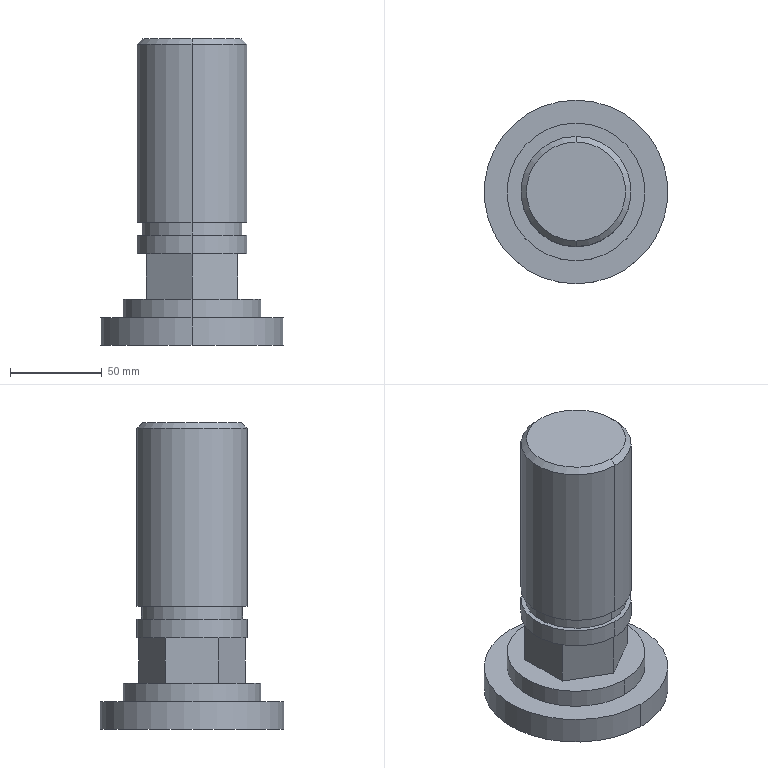Component | SolidWorks | ConnectingRod-1 | 1 solid | 25 faces | box 100 x 100 x 167 mm | volume 542943 mm3 | plane 13 | cylinder 10 | cone 2 | commonest cylinder face diameters 60 x4 55 x2 75 x2 100 x2
build123d program:
from build123d import *

# Parameters (mm, degrees)
SKETCH1_W           = 50
SKETCH1_H           = 15
SKETCH2_R           = 37.5
BOSS_EXTRUDE1_DEPTH = 10
BOSS_EXTRUDE2_DEPTH = 25
SKETCH4_R           = 30
BOSS_EXTRUDE3_DEPTH = 10
SKETCH5_R           = 27.5
BOSS_EXTRUDE4_DEPTH = 7
SKETCH6_R           = 30
BOSS_EXTRUDE5_DEPTH = 100
CHAMFER1_SIZE       = 3
CHAMFER1_SIZE2      = 3


with BuildPart() as part:
    # Sketch1 → Revolve1 (revolve)
    with BuildSketch(Plane(origin=(0, 0, 0), x_dir=(1, 0, 0), z_dir=(0, 1, 0))):
        with Locations((25, 12.5)):
            Rectangle(SKETCH1_W, SKETCH1_H)
    revolve(axis=Axis((0, 0, -20), (0, 0, 1)))

    # Sketch2 → Boss-Extrude1 (add)
    with BuildSketch(Plane.XY.offset(-5)):
        Circle(SKETCH2_R)
    extrude(amount=BOSS_EXTRUDE1_DEPTH)

    # Sketch3 → Boss-Extrude2 (add)
    with BuildSketch(Plane.XY.offset(5)):
        Polygon((28.868, 0), (14.434, -25), (-14.434, -25), (-28.868, 0), (-14.434, 25), (14.434, 25), align=None)
    extrude(amount=BOSS_EXTRUDE2_DEPTH)

    # Sketch4 → Boss-Extrude3 (add)
    with BuildSketch(Plane(origin=(0, 0, 30), x_dir=(-1, 0, 0), z_dir=(0, 0, -1))):
        with Locations(Location((0, 0, 0), (0, 0, 180))):
            Circle(SKETCH4_R)
    extrude(amount=-BOSS_EXTRUDE3_DEPTH)

    # Sketch5 → Boss-Extrude4 (add)
    with BuildSketch(Plane.XY.offset(40)):
        with Locations(Location((0, 0, 0), (0, 0, 180))):
            Circle(SKETCH5_R)
    extrude(amount=BOSS_EXTRUDE4_DEPTH)

    # Sketch6 → Boss-Extrude5 (add)
    with BuildSketch(Plane(origin=(0, 0, 47), x_dir=(-1, 0, 0), z_dir=(0, 0, -1))):
        with Locations(Location((0, 0, 0), (0, 0, 180))):
            Circle(SKETCH6_R)
    extrude(amount=-BOSS_EXTRUDE5_DEPTH)

    # Chamfer1
    chamfer1_edges = [part.edges().sort_by_distance(p)[0] for p in [
        (-30, 0, 147),
    ]]
    chamfer1_side = [part.faces().sort_by_distance(p)[0] for p in [
        (-30, 0, 97),
    ]]
    chamfer(chamfer1_edges, length=CHAMFER1_SIZE, length2=CHAMFER1_SIZE2, reference=chamfer1_side[0])


solid = part.part

# Placed as in the assembly
solid = solid.moved(Location((-505.158, 870.769, 834.663), (0, 0, 90)))
STEP:
#1=COLOUR_RGB('',0.7922,0.8196,0.9333);
#2=FILL_AREA_STYLE_COLOUR('',#1);
#3=FILL_AREA_STYLE('',(#2));
#4=SURFACE_STYLE_FILL_AREA(#3);
#5=SURFACE_SIDE_STYLE('',(#4));
#6=SURFACE_STYLE_USAGE(.BOTH.,#5);
#7=PRESENTATION_STYLE_ASSIGNMENT((#6));
#8=CARTESIAN_POINT('',(-19.888,35.345,38.648));
#9=VERTEX_POINT('',#8);
#10=CARTESIAN_POINT('',(-19.888,33.219,38.648));
#11=VERTEX_POINT('',#10);
#12=CARTESIAN_POINT('',(-19.888,34.282,38.648));
#13=DIRECTION('',(0.,0.,1.));
#14=DIRECTION('',(0.,1.,0.));
#15=AXIS2_PLACEMENT_3D('',#12,#13,#14);
#16=CIRCLE('',#15,1.063);
#17=EDGE_CURVE('',#9,#11,#16,.T.);
#18=ORIENTED_EDGE('',*,*,#17,.F.);
#19=CARTESIAN_POINT('',(-19.888,35.463,38.53));
#20=VERTEX_POINT('',#19);
#21=CARTESIAN_POINT('',(-19.888,35.463,38.53));
#22=DIRECTION('',(-0.,0.7071,-0.7071));
#23=VECTOR('',#22,39.37);
#24=LINE('',#21,#23);
#25=EDGE_CURVE('',#9,#20,#24,.T.);
#26=ORIENTED_EDGE('',*,*,#25,.T.);
#27=CARTESIAN_POINT('',(-19.888,33.101,38.53));
#28=VERTEX_POINT('',#27);
#29=CARTESIAN_POINT('',(-19.888,34.282,38.53));
#30=DIRECTION('',(0.,0.,-1.));
#31=DIRECTION('',(0.,1.,0.));
#32=AXIS2_PLACEMENT_3D('',#29,#30,#31);
#33=CIRCLE('',#32,1.181);
#34=EDGE_CURVE('',#28,#20,#33,.T.);
#35=ORIENTED_EDGE('',*,*,#34,.F.);
#36=CARTESIAN_POINT('',(-19.888,33.101,38.53));
#37=DIRECTION('',(0.,-0.7071,-0.7071));
#38=VECTOR('',#37,39.37);
#39=LINE('',#36,#38);
#40=EDGE_CURVE('',#11,#28,#39,.T.);
#41=ORIENTED_EDGE('',*,*,#40,.F.);
#42=EDGE_LOOP('',(#18,#26,#35,#41));
#43=FACE_OUTER_BOUND('',#42,.T.);
#44=CARTESIAN_POINT('',(-19.888,34.282,38.53));
#45=DIRECTION('',(0.,0.,-1.));
#46=DIRECTION('',(0.,-1.,0.));
#47=AXIS2_PLACEMENT_3D('',#44,#45,#46);
#48=CONICAL_SURFACE('',#47,1.181,0.7854);
#49=ADVANCED_FACE('',(#43),#48,.T.);
#50=ORIENTED_EDGE('',*,*,#34,.T.);
#51=CARTESIAN_POINT('',(-19.888,35.463,34.711));
#52=VERTEX_POINT('',#51);
#53=CARTESIAN_POINT('',(-19.888,35.463,38.648));
#54=DIRECTION('',(0.,0.,-1.));
#55=VECTOR('',#54,39.37);
#56=LINE('',#53,#55);
#57=EDGE_CURVE('',#20,#52,#56,.T.);
#58=ORIENTED_EDGE('',*,*,#57,.T.);
#59=CARTESIAN_POINT('',(-19.888,33.101,34.711));
#60=VERTEX_POINT('',#59);
#61=CARTESIAN_POINT('',(-19.888,34.282,34.711));
#62=DIRECTION('',(0.,0.,-1.));
#63=DIRECTION('',(0.,1.,0.));
#64=AXIS2_PLACEMENT_3D('',#61,#62,#63);
#65=CIRCLE('',#64,1.181);
#66=EDGE_CURVE('',#60,#52,#65,.T.);
#67=ORIENTED_EDGE('',*,*,#66,.F.);
#68=CARTESIAN_POINT('',(-19.888,33.101,38.648));
#69=DIRECTION('',(0.,0.,-1.));
#70=VECTOR('',#69,39.37);
#71=LINE('',#68,#70);
#72=EDGE_CURVE('',#28,#60,#71,.T.);
#73=ORIENTED_EDGE('',*,*,#72,.F.);
#74=EDGE_LOOP('',(#50,#58,#67,#73));
#75=FACE_OUTER_BOUND('',#74,.T.);
#76=CARTESIAN_POINT('',(-19.888,34.282,38.648));
#77=DIRECTION('',(0.,0.,-1.));
#78=DIRECTION('',(0.,-1.,0.));
#79=AXIS2_PLACEMENT_3D('',#76,#77,#78);
#80=CYLINDRICAL_SURFACE('',#79,1.181);
#81=ADVANCED_FACE('',(#75),#80,.T.);
#82=CARTESIAN_POINT('',(-19.888,35.365,34.711));
#83=VERTEX_POINT('',#82);
#84=CARTESIAN_POINT('',(-19.888,33.2,34.711));
#85=VERTEX_POINT('',#84);
#86=CARTESIAN_POINT('',(-19.888,34.282,34.711));
#87=DIRECTION('',(0.,0.,1.));
#88=DIRECTION('',(0.,1.,0.));
#89=AXIS2_PLACEMENT_3D('',#86,#87,#88);
#90=CIRCLE('',#89,1.083);
#91=EDGE_CURVE('',#83,#85,#90,.T.);
#92=ORIENTED_EDGE('',*,*,#91,.F.);
#93=CARTESIAN_POINT('',(-19.888,35.365,34.436));
#94=VERTEX_POINT('',#93);
#95=CARTESIAN_POINT('',(-19.888,35.365,34.711));
#96=DIRECTION('',(0.,0.,-1.));
#97=VECTOR('',#96,39.37);
#98=LINE('',#95,#97);
#99=EDGE_CURVE('',#83,#94,#98,.T.);
#100=ORIENTED_EDGE('',*,*,#99,.T.);
#101=CARTESIAN_POINT('',(-19.888,33.2,34.436));
#102=VERTEX_POINT('',#101);
#103=CARTESIAN_POINT('',(-19.888,34.282,34.436));
#104=DIRECTION('',(0.,0.,1.));
#105=DIRECTION('',(0.,1.,0.));
#106=AXIS2_PLACEMENT_3D('',#103,#104,#105);
#107=CIRCLE('',#106,1.083);
#108=EDGE_CURVE('',#94,#102,#107,.T.);
#109=ORIENTED_EDGE('',*,*,#108,.T.);
#110=CARTESIAN_POINT('',(-19.888,33.2,34.711));
#111=DIRECTION('',(0.,0.,-1.));
#112=VECTOR('',#111,39.37);
#113=LINE('',#110,#112);
#114=EDGE_CURVE('',#85,#102,#113,.T.);
#115=ORIENTED_EDGE('',*,*,#114,.F.);
#116=EDGE_LOOP('',(#92,#100,#109,#115));
#117=FACE_OUTER_BOUND('',#116,.T.);
#118=CARTESIAN_POINT('',(-19.888,34.282,34.711));
#119=DIRECTION('',(0.,0.,-1.));
#120=DIRECTION('',(0.,-1.,0.));
#121=AXIS2_PLACEMENT_3D('',#118,#119,#120);
#122=CYLINDRICAL_SURFACE('',#121,1.083);
#123=ADVANCED_FACE('',(#117),#122,.T.);
#124=CARTESIAN_POINT('',(-19.888,33.101,34.436));
#125=VERTEX_POINT('',#124);
#126=CARTESIAN_POINT('',(-19.888,35.463,34.436));
#127=VERTEX_POINT('',#126);
#128=CARTESIAN_POINT('',(-19.888,34.282,34.436));
#129=DIRECTION('',(0.,0.,-1.));
#130=DIRECTION('',(0.,1.,0.));
#131=AXIS2_PLACEMENT_3D('',#128,#129,#130);
#132=CIRCLE('',#131,1.181);
#133=EDGE_CURVE('',#125,#127,#132,.T.);
#134=ORIENTED_EDGE('',*,*,#133,.T.);
#135=CARTESIAN_POINT('',(-19.888,35.463,34.042));
#136=VERTEX_POINT('',#135);
#137=CARTESIAN_POINT('',(-19.888,35.463,34.436));
#138=DIRECTION('',(0.,0.,-1.));
#139=VECTOR('',#138,39.37);
#140=LINE('',#137,#139);
#141=EDGE_CURVE('',#127,#136,#140,.T.);
#142=ORIENTED_EDGE('',*,*,#141,.T.);
#143=CARTESIAN_POINT('',(-19.888,33.101,34.042));
#144=VERTEX_POINT('',#143);
#145=CARTESIAN_POINT('',(-19.888,34.282,34.042));
#146=DIRECTION('',(0.,0.,-1.));
#147=DIRECTION('',(0.,1.,0.));
#148=AXIS2_PLACEMENT_3D('',#145,#146,#147);
#149=CIRCLE('',#148,1.181);
#150=EDGE_CURVE('',#144,#136,#149,.T.);
#151=ORIENTED_EDGE('',*,*,#150,.F.);
#152=CARTESIAN_POINT('',(-19.888,33.101,34.436));
#153=DIRECTION('',(0.,0.,-1.));
#154=VECTOR('',#153,39.37);
#155=LINE('',#152,#154);
#156=EDGE_CURVE('',#125,#144,#155,.T.);
#157=ORIENTED_EDGE('',*,*,#156,.F.);
#158=EDGE_LOOP('',(#134,#142,#151,#157));
#159=FACE_OUTER_BOUND('',#158,.T.);
#160=CARTESIAN_POINT('',(-19.888,34.282,34.436));
#161=DIRECTION('',(0.,0.,-1.));
#162=DIRECTION('',(0.,-1.,0.));
#163=AXIS2_PLACEMENT_3D('',#160,#161,#162);
#164=CYLINDRICAL_SURFACE('',#163,1.181);
#165=ADVANCED_FACE('',(#159),#164,.T.);
#166=CARTESIAN_POINT('',(-19.888,35.759,33.058));
#167=VERTEX_POINT('',#166);
#168=CARTESIAN_POINT('',(-19.888,32.806,33.058));
#169=VERTEX_POINT('',#168);
#170=CARTESIAN_POINT('',(-19.888,34.282,33.058));
#171=DIRECTION('',(0.,0.,1.));
#172=DIRECTION('',(0.,1.,0.));
#173=AXIS2_PLACEMENT_3D('',#170,#171,#172);
#174=CIRCLE('',#173,1.476);
#175=EDGE_CURVE('',#167,#169,#174,.T.);
#176=ORIENTED_EDGE('',*,*,#175,.F.);
#177=CARTESIAN_POINT('',(-19.888,35.759,32.664));
#178=VERTEX_POINT('',#177);
#179=CARTESIAN_POINT('',(-19.888,35.759,33.058));
#180=DIRECTION('',(0.,0.,-1.));
#181=VECTOR('',#180,39.37);
#182=LINE('',#179,#181);
#183=EDGE_CURVE('',#167,#178,#182,.T.);
#184=ORIENTED_EDGE('',*,*,#183,.T.);
#185=CARTESIAN_POINT('',(-19.888,32.806,32.664));
#186=VERTEX_POINT('',#185);
#187=CARTESIAN_POINT('',(-19.888,34.282,32.664));
#188=DIRECTION('',(0.,0.,1.));
#189=DIRECTION('',(0.,1.,0.));
#190=AXIS2_PLACEMENT_3D('',#187,#188,#189);
#191=CIRCLE('',#190,1.476);
#192=EDGE_CURVE('',#178,#186,#191,.T.);
#193=ORIENTED_EDGE('',*,*,#192,.T.);
#194=CARTESIAN_POINT('',(-19.888,32.806,33.058));
#195=DIRECTION('',(0.,0.,-1.));
#196=VECTOR('',#195,39.37);
#197=LINE('',#194,#196);
#198=EDGE_CURVE('',#169,#186,#197,.T.);
#199=ORIENTED_EDGE('',*,*,#198,.F.);
#200=EDGE_LOOP('',(#176,#184,#193,#199));
#201=FACE_OUTER_BOUND('',#200,.T.);
#202=CARTESIAN_POINT('',(-19.888,34.282,33.058));
#203=DIRECTION('',(0.,0.,-1.));
#204=DIRECTION('',(0.,-1.,0.));
#205=AXIS2_PLACEMENT_3D('',#202,#203,#204);
#206=CYLINDRICAL_SURFACE('',#205,1.476);
#207=ADVANCED_FACE('',(#201),#206,.T.);
#208=CARTESIAN_POINT('',(-19.888,36.251,32.073));
#209=VERTEX_POINT('',#208);
#210=CARTESIAN_POINT('',(-19.888,32.314,32.073));
#211=VERTEX_POINT('',#210);
#212=CARTESIAN_POINT('',(-19.888,34.282,32.073));
#213=DIRECTION('',(0.,0.,1.));
#214=DIRECTION('',(0.,1.,0.));
#215=AXIS2_PLACEMENT_3D('',#212,#213,#214);
#216=CIRCLE('',#215,1.969);
#217=EDGE_CURVE('',#209,#211,#216,.T.);
#218=ORIENTED_EDGE('',*,*,#217,.T.);
#219=CARTESIAN_POINT('',(-19.888,32.314,32.664));
#220=VERTEX_POINT('',#219);
#221=CARTESIAN_POINT('',(-19.888,32.314,32.073));
#222=DIRECTION('',(0.,0.,1.));
#223=VECTOR('',#222,39.37);
#224=LINE('',#221,#223);
#225=EDGE_CURVE('',#211,#220,#224,.T.);
#226=ORIENTED_EDGE('',*,*,#225,.T.);
#227=CARTESIAN_POINT('',(-19.888,36.251,32.664));
#228=VERTEX_POINT('',#227);
#229=CARTESIAN_POINT('',(-19.888,34.282,32.664));
#230=DIRECTION('',(0.,0.,1.));
#231=DIRECTION('',(0.,1.,0.));
#232=AXIS2_PLACEMENT_3D('',#229,#230,#231);
#233=CIRCLE('',#232,1.969);
#234=EDGE_CURVE('',#228,#220,#233,.T.);
#235=ORIENTED_EDGE('',*,*,#234,.F.);
#236=CARTESIAN_POINT('',(-19.888,36.251,32.073));
#237=DIRECTION('',(0.,0.,1.));
#238=VECTOR('',#237,39.37);
#239=LINE('',#236,#238);
#240=EDGE_CURVE('',#209,#228,#239,.T.);
#241=ORIENTED_EDGE('',*,*,#240,.F.);
#242=EDGE_LOOP('',(#218,#226,#235,#241));
#243=FACE_OUTER_BOUND('',#242,.T.);
#244=CARTESIAN_POINT('',(-19.888,34.282,32.073));
#245=DIRECTION('',(0.,0.,1.));
#246=DIRECTION('',(0.,1.,0.));
#247=AXIS2_PLACEMENT_3D('',#244,#245,#246);
#248=CYLINDRICAL_SURFACE('',#247,1.969);
#249=ADVANCED_FACE('',(#243),#248,.T.);
#250=ORIENTED_EDGE('',*,*,#225,.F.);
#251=CARTESIAN_POINT('',(-19.888,34.282,32.073));
#252=DIRECTION('',(0.,0.,1.));
#253=DIRECTION('',(0.,1.,0.));
#254=AXIS2_PLACEMENT_3D('',#251,#252,#253);
#255=CIRCLE('',#254,1.969);
#256=EDGE_CURVE('',#211,#209,#255,.T.);
#257=ORIENTED_EDGE('',*,*,#256,.T.);
#258=ORIENTED_EDGE('',*,*,#240,.T.);
#259=CARTESIAN_POINT('',(-19.888,34.282,32.664));
#260=DIRECTION('',(0.,0.,1.));
#261=DIRECTION('',(0.,1.,0.));
#262=AXIS2_PLACEMENT_3D('',#259,#260,#261);
#263=CIRCLE('',#262,1.969);
#264=EDGE_CURVE('',#220,#228,#263,.T.);
#265=ORIENTED_EDGE('',*,*,#264,.F.);
#266=EDGE_LOOP('',(#250,#257,#258,#265));
#267=FACE_OUTER_BOUND('',#266,.T.);
#268=CARTESIAN_POINT('',(-19.888,34.282,32.073));
#269=DIRECTION('',(0.,0.,1.));
#270=DIRECTION('',(0.,1.,0.));
#271=AXIS2_PLACEMENT_3D('',#268,#269,#270);
#272=CYLINDRICAL_SURFACE('',#271,1.969);
#273=ADVANCED_FACE('',(#267),#272,.T.);
#274=ORIENTED_EDGE('',*,*,#217,.F.);
#275=ORIENTED_EDGE('',*,*,#256,.F.);
#276=EDGE_LOOP('',(#274,#275));
#277=FACE_OUTER_BOUND('',#276,.T.);
#278=CARTESIAN_POINT('',(-19.888,36.251,32.073));
#279=DIRECTION('',(0.,0.,-1.));
#280=DIRECTION('',(0.,-1.,0.));
#281=AXIS2_PLACEMENT_3D('',#278,#279,#280);
#282=PLANE('',#281);
#283=ADVANCED_FACE('',(#277),#282,.T.);
#284=CARTESIAN_POINT('',(-19.888,34.282,32.664));
#285=DIRECTION('',(0.,0.,1.));
#286=DIRECTION('',(0.,1.,0.));
#287=AXIS2_PLACEMENT_3D('',#284,#285,#286);
#288=CIRCLE('',#287,1.476);
#289=EDGE_CURVE('',#186,#178,#288,.T.);
#290=ORIENTED_EDGE('',*,*,#289,.F.);
#291=ORIENTED_EDGE('',*,*,#192,.F.);
#292=EDGE_LOOP('',(#290,#291));
#293=FACE_BOUND('',#292,.T.);
#294=ORIENTED_EDGE('',*,*,#234,.T.);
#295=ORIENTED_EDGE('',*,*,#264,.T.);
#296=EDGE_LOOP('',(#294,#295));
#297=FACE_OUTER_BOUND('',#296,.T.);
#298=CARTESIAN_POINT('',(-19.888,34.282,32.664));
#299=DIRECTION('',(0.,0.,1.));
#300=DIRECTION('',(0.,1.,0.));
#301=AXIS2_PLACEMENT_3D('',#298,#299,#300);
#302=PLANE('',#301);
#303=ADVANCED_FACE('',(#293,#297),#302,.T.);
#304=ORIENTED_EDGE('',*,*,#183,.F.);
#305=CARTESIAN_POINT('',(-19.888,34.282,33.058));
#306=DIRECTION('',(0.,0.,1.));
#307=DIRECTION('',(0.,1.,0.));
#308=AXIS2_PLACEMENT_3D('',#305,#306,#307);
#309=CIRCLE('',#308,1.476);
#310=EDGE_CURVE('',#169,#167,#309,.T.);
#311=ORIENTED_EDGE('',*,*,#310,.F.);
#312=ORIENTED_EDGE('',*,*,#198,.T.);
#313=ORIENTED_EDGE('',*,*,#289,.T.);
#314=EDGE_LOOP('',(#304,#311,#312,#313));
#315=FACE_OUTER_BOUND('',#314,.T.);
#316=CARTESIAN_POINT('',(-19.888,34.282,33.058));
#317=DIRECTION('',(0.,0.,-1.));
#318=DIRECTION('',(0.,-1.,0.));
#319=AXIS2_PLACEMENT_3D('',#316,#317,#318);
#320=CYLINDRICAL_SURFACE('',#319,1.476);
#321=ADVANCED_FACE('',(#315),#320,.T.);
#322=CARTESIAN_POINT('',(-19.888,35.419,33.058));
#323=VERTEX_POINT('',#322);
#324=CARTESIAN_POINT('',(-20.872,34.85,33.058));
#325=VERTEX_POINT('',#324);
#326=CARTESIAN_POINT('',(-20.872,34.85,33.058));
#327=DIRECTION('',(-0.866,-0.5,0.));
#328=VECTOR('',#327,39.37);
#329=LINE('',#326,#328);
#330=EDGE_CURVE('',#323,#325,#329,.T.);
#331=ORIENTED_EDGE('',*,*,#330,.F.);
#332=CARTESIAN_POINT('',(-18.904,34.85,33.058));
#333=VERTEX_POINT('',#332);
#334=CARTESIAN_POINT('',(-19.888,35.419,33.058));
#335=DIRECTION('',(-0.866,0.5,0.));
#336=VECTOR('',#335,39.37);
#337=LINE('',#334,#336);
#338=EDGE_CURVE('',#333,#323,#337,.T.);
#339=ORIENTED_EDGE('',*,*,#338,.F.);
#340=CARTESIAN_POINT('',(-18.904,33.714,33.058));
#341=VERTEX_POINT('',#340);
#342=CARTESIAN_POINT('',(-18.904,34.85,33.058));
#343=DIRECTION('',(0.,1.,0.));
#344=VECTOR('',#343,39.37);
#345=LINE('',#342,#344);
#346=EDGE_CURVE('',#341,#333,#345,.T.);
#347=ORIENTED_EDGE('',*,*,#346,.F.);
#348=CARTESIAN_POINT('',(-19.888,33.146,33.058));
#349=VERTEX_POINT('',#348);
#350=CARTESIAN_POINT('',(-18.904,33.714,33.058));
#351=DIRECTION('',(0.866,0.5,0.));
#352=VECTOR('',#351,39.37);
#353=LINE('',#350,#352);
#354=EDGE_CURVE('',#349,#341,#353,.T.);
#355=ORIENTED_EDGE('',*,*,#354,.F.);
#356=CARTESIAN_POINT('',(-20.872,33.714,33.058));
#357=VERTEX_POINT('',#356);
#358=CARTESIAN_POINT('',(-19.888,33.146,33.058));
#359=DIRECTION('',(0.866,-0.5,0.));
#360=VECTOR('',#359,39.37);
#361=LINE('',#358,#360);
#362=EDGE_CURVE('',#357,#349,#361,.T.);
#363=ORIENTED_EDGE('',*,*,#362,.F.);
#364=CARTESIAN_POINT('',(-20.872,33.714,33.058));
#365=DIRECTION('',(0.,-1.,0.));
#366=VECTOR('',#365,39.37);
#367=LINE('',#364,#366);
#368=EDGE_CURVE('',#325,#357,#367,.T.);
#369=ORIENTED_EDGE('',*,*,#368,.F.);
#370=EDGE_LOOP('',(#331,#339,#347,#355,#363,#369));
#371=FACE_BOUND('',#370,.T.);
#372=ORIENTED_EDGE('',*,*,#310,.T.);
#373=ORIENTED_EDGE('',*,*,#175,.T.);
#374=EDGE_LOOP('',(#372,#373));
#375=FACE_OUTER_BOUND('',#374,.T.);
#376=CARTESIAN_POINT('',(-19.888,34.282,33.058));
#377=DIRECTION('',(0.,0.,1.));
#378=DIRECTION('',(0.,1.,0.));
#379=AXIS2_PLACEMENT_3D('',#376,#377,#378);
#380=PLANE('',#379);
#381=ADVANCED_FACE('',(#371,#375),#380,.T.);
#382=ORIENTED_EDGE('',*,*,#330,.T.);
#383=CARTESIAN_POINT('',(-20.872,34.85,34.042));
#384=VERTEX_POINT('',#383);
#385=CARTESIAN_POINT('',(-20.872,34.85,34.042));
#386=DIRECTION('',(0.,0.,-1.));
#387=VECTOR('',#386,39.37);
#388=LINE('',#385,#387);
#389=EDGE_CURVE('',#384,#325,#388,.T.);
#390=ORIENTED_EDGE('',*,*,#389,.F.);
#391=CARTESIAN_POINT('',(-19.888,35.419,34.042));
#392=VERTEX_POINT('',#391);
#393=CARTESIAN_POINT('',(-20.872,34.85,34.042));
#394=DIRECTION('',(-0.866,-0.5,0.));
#395=VECTOR('',#394,39.37);
#396=LINE('',#393,#395);
#397=EDGE_CURVE('',#392,#384,#396,.T.);
#398=ORIENTED_EDGE('',*,*,#397,.F.);
#399=CARTESIAN_POINT('',(-19.888,35.419,34.042));
#400=DIRECTION('',(0.,0.,-1.));
#401=VECTOR('',#400,39.37);
#402=LINE('',#399,#401);
#403=EDGE_CURVE('',#392,#323,#402,.T.);
#404=ORIENTED_EDGE('',*,*,#403,.T.);
#405=EDGE_LOOP('',(#382,#390,#398,#404));
#406=FACE_OUTER_BOUND('',#405,.T.);
#407=CARTESIAN_POINT('',(-20.872,34.85,34.042));
#408=DIRECTION('',(0.5,-0.866,0.));
#409=DIRECTION('',(0.866,0.5,0.));
#410=AXIS2_PLACEMENT_3D('',#407,#408,#409);
#411=PLANE('',#410);
#412=ADVANCED_FACE('',(#406),#411,.F.);
#413=ORIENTED_EDGE('',*,*,#368,.T.);
#414=CARTESIAN_POINT('',(-20.872,33.714,34.042));
#415=VERTEX_POINT('',#414);
#416=CARTESIAN_POINT('',(-20.872,33.714,34.042));
#417=DIRECTION('',(0.,0.,-1.));
#418=VECTOR('',#417,39.37);
#419=LINE('',#416,#418);
#420=EDGE_CURVE('',#415,#357,#419,.T.);
#421=ORIENTED_EDGE('',*,*,#420,.F.);
#422=CARTESIAN_POINT('',(-20.872,33.714,34.042));
#423=DIRECTION('',(0.,-1.,0.));
#424=VECTOR('',#423,39.37);
#425=LINE('',#422,#424);
#426=EDGE_CURVE('',#384,#415,#425,.T.);
#427=ORIENTED_EDGE('',*,*,#426,.F.);
#428=ORIENTED_EDGE('',*,*,#389,.T.);
#429=EDGE_LOOP('',(#413,#421,#427,#428));
#430=FACE_OUTER_BOUND('',#429,.T.);
#431=CARTESIAN_POINT('',(-20.872,33.714,34.042));
#432=DIRECTION('',(1.,0.,0.));
#433=DIRECTION('',(0.,0.,-1.));
#434=AXIS2_PLACEMENT_3D('',#431,#432,#433);
#435=PLANE('',#434);
#436=ADVANCED_FACE('',(#430),#435,.F.);
#437=ORIENTED_EDGE('',*,*,#362,.T.);
#438=CARTESIAN_POINT('',(-19.888,33.146,34.042));
#439=VERTEX_POINT('',#438);
#440=CARTESIAN_POINT('',(-19.888,33.146,34.042));
#441=DIRECTION('',(0.,0.,-1.));
#442=VECTOR('',#441,39.37);
#443=LINE('',#440,#442);
#444=EDGE_CURVE('',#439,#349,#443,.T.);
#445=ORIENTED_EDGE('',*,*,#444,.F.);
#446=CARTESIAN_POINT('',(-19.888,33.146,34.042));
#447=DIRECTION('',(0.866,-0.5,0.));
#448=VECTOR('',#447,39.37);
#449=LINE('',#446,#448);
#450=EDGE_CURVE('',#415,#439,#449,.T.);
#451=ORIENTED_EDGE('',*,*,#450,.F.);
#452=ORIENTED_EDGE('',*,*,#420,.T.);
#453=EDGE_LOOP('',(#437,#445,#451,#452));
#454=FACE_OUTER_BOUND('',#453,.T.);
#455=CARTESIAN_POINT('',(-19.888,33.146,34.042));
#456=DIRECTION('',(0.5,0.866,0.));
#457=DIRECTION('',(-0.866,0.5,0.));
#458=AXIS2_PLACEMENT_3D('',#455,#456,#457);
#459=PLANE('',#458);
#460=ADVANCED_FACE('',(#454),#459,.F.);
#461=ORIENTED_EDGE('',*,*,#354,.T.);
#462=CARTESIAN_POINT('',(-18.904,33.714,34.042));
#463=VERTEX_POINT('',#462);
#464=CARTESIAN_POINT('',(-18.904,33.714,34.042));
#465=DIRECTION('',(0.,0.,-1.));
#466=VECTOR('',#465,39.37);
#467=LINE('',#464,#466);
#468=EDGE_CURVE('',#463,#341,#467,.T.);
#469=ORIENTED_EDGE('',*,*,#468,.F.);
#470=CARTESIAN_POINT('',(-18.904,33.714,34.042));
#471=DIRECTION('',(0.866,0.5,0.));
#472=VECTOR('',#471,39.37);
#473=LINE('',#470,#472);
#474=EDGE_CURVE('',#439,#463,#473,.T.);
#475=ORIENTED_EDGE('',*,*,#474,.F.);
#476=ORIENTED_EDGE('',*,*,#444,.T.);
#477=EDGE_LOOP('',(#461,#469,#475,#476));
#478=FACE_OUTER_BOUND('',#477,.T.);
#479=CARTESIAN_POINT('',(-18.904,33.714,34.042));
#480=DIRECTION('',(-0.5,0.866,0.));
#481=DIRECTION('',(-0.866,-0.5,0.));
#482=AXIS2_PLACEMENT_3D('',#479,#480,#481);
#483=PLANE('',#482);
#484=ADVANCED_FACE('',(#478),#483,.F.);
#485=ORIENTED_EDGE('',*,*,#346,.T.);
#486=CARTESIAN_POINT('',(-18.904,34.85,34.042));
#487=VERTEX_POINT('',#486);
#488=CARTESIAN_POINT('',(-18.904,34.85,34.042));
#489=DIRECTION('',(0.,0.,-1.));
#490=VECTOR('',#489,39.37);
#491=LINE('',#488,#490);
#492=EDGE_CURVE('',#487,#333,#491,.T.);
#493=ORIENTED_EDGE('',*,*,#492,.F.);
#494=CARTESIAN_POINT('',(-18.904,34.85,34.042));
#495=DIRECTION('',(0.,1.,0.));
#496=VECTOR('',#495,39.37);
#497=LINE('',#494,#496);
#498=EDGE_CURVE('',#463,#487,#497,.T.);
#499=ORIENTED_EDGE('',*,*,#498,.F.);
#500=ORIENTED_EDGE('',*,*,#468,.T.);
#501=EDGE_LOOP('',(#485,#493,#499,#500));
#502=FACE_OUTER_BOUND('',#501,.T.);
#503=CARTESIAN_POINT('',(-18.904,34.85,34.042));
#504=DIRECTION('',(-1.,0.,0.));
#505=DIRECTION('',(-0.,-1.,0.));
#506=AXIS2_PLACEMENT_3D('',#503,#504,#505);
#507=PLANE('',#506);
#508=ADVANCED_FACE('',(#502),#507,.F.);
#509=ORIENTED_EDGE('',*,*,#338,.T.);
#510=ORIENTED_EDGE('',*,*,#403,.F.);
#511=CARTESIAN_POINT('',(-19.888,35.419,34.042));
#512=DIRECTION('',(-0.866,0.5,0.));
#513=VECTOR('',#512,39.37);
#514=LINE('',#511,#513);
#515=EDGE_CURVE('',#487,#392,#514,.T.);
#516=ORIENTED_EDGE('',*,*,#515,.F.);
#517=ORIENTED_EDGE('',*,*,#492,.T.);
#518=EDGE_LOOP('',(#509,#510,#516,#517));
#519=FACE_OUTER_BOUND('',#518,.T.);
#520=CARTESIAN_POINT('',(-19.888,35.419,34.042));
#521=DIRECTION('',(-0.5,-0.866,0.));
#522=DIRECTION('',(0.866,-0.5,0.));
#523=AXIS2_PLACEMENT_3D('',#520,#521,#522);
#524=PLANE('',#523);
#525=ADVANCED_FACE('',(#519),#524,.F.);
#526=ORIENTED_EDGE('',*,*,#150,.T.);
#527=CARTESIAN_POINT('',(-19.888,34.282,34.042));
#528=DIRECTION('',(0.,0.,-1.));
#529=DIRECTION('',(0.,1.,0.));
#530=AXIS2_PLACEMENT_3D('',#527,#528,#529);
#531=CIRCLE('',#530,1.181);
#532=EDGE_CURVE('',#136,#144,#531,.T.);
#533=ORIENTED_EDGE('',*,*,#532,.T.);
#534=EDGE_LOOP('',(#526,#533));
#535=FACE_OUTER_BOUND('',#534,.T.);
#536=ORIENTED_EDGE('',*,*,#515,.T.);
#537=ORIENTED_EDGE('',*,*,#397,.T.);
#538=ORIENTED_EDGE('',*,*,#426,.T.);
#539=ORIENTED_EDGE('',*,*,#450,.T.);
#540=ORIENTED_EDGE('',*,*,#474,.T.);
#541=ORIENTED_EDGE('',*,*,#498,.T.);
#542=EDGE_LOOP('',(#536,#537,#538,#539,#540,#541));
#543=FACE_BOUND('',#542,.T.);
#544=CARTESIAN_POINT('',(-19.888,34.282,34.042));
#545=DIRECTION('',(0.,0.,1.));
#546=DIRECTION('',(0.,1.,0.));
#547=AXIS2_PLACEMENT_3D('',#544,#545,#546);
#548=PLANE('',#547);
#549=ADVANCED_FACE('',(#535,#543),#548,.F.);
#550=ORIENTED_EDGE('',*,*,#141,.F.);
#551=CARTESIAN_POINT('',(-19.888,34.282,34.436));
#552=DIRECTION('',(0.,0.,-1.));
#553=DIRECTION('',(0.,1.,0.));
#554=AXIS2_PLACEMENT_3D('',#551,#552,#553);
#555=CIRCLE('',#554,1.181);
#556=EDGE_CURVE('',#127,#125,#555,.T.);
#557=ORIENTED_EDGE('',*,*,#556,.T.);
#558=ORIENTED_EDGE('',*,*,#156,.T.);
#559=ORIENTED_EDGE('',*,*,#532,.F.);
#560=EDGE_LOOP('',(#550,#557,#558,#559));
#561=FACE_OUTER_BOUND('',#560,.T.);
#562=CARTESIAN_POINT('',(-19.888,34.282,34.436));
#563=DIRECTION('',(0.,0.,-1.));
#564=DIRECTION('',(0.,-1.,0.));
#565=AXIS2_PLACEMENT_3D('',#562,#563,#564);
#566=CYLINDRICAL_SURFACE('',#565,1.181);
#567=ADVANCED_FACE('',(#561),#566,.T.);
#568=CARTESIAN_POINT('',(-19.888,34.282,34.436));
#569=DIRECTION('',(0.,0.,1.));
#570=DIRECTION('',(0.,1.,0.));
#571=AXIS2_PLACEMENT_3D('',#568,#569,#570);
#572=CIRCLE('',#571,1.083);
#573=EDGE_CURVE('',#102,#94,#572,.T.);
#574=ORIENTED_EDGE('',*,*,#573,.F.);
#575=ORIENTED_EDGE('',*,*,#108,.F.);
#576=EDGE_LOOP('',(#574,#575));
#577=FACE_BOUND('',#576,.T.);
#578=ORIENTED_EDGE('',*,*,#133,.F.);
#579=ORIENTED_EDGE('',*,*,#556,.F.);
#580=EDGE_LOOP('',(#578,#579));
#581=FACE_OUTER_BOUND('',#580,.T.);
#582=CARTESIAN_POINT('',(-19.888,34.282,34.436));
#583=DIRECTION('',(0.,0.,1.));
#584=DIRECTION('',(0.,1.,0.));
#585=AXIS2_PLACEMENT_3D('',#582,#583,#584);
#586=PLANE('',#585);
#587=ADVANCED_FACE('',(#577,#581),#586,.T.);
#588=ORIENTED_EDGE('',*,*,#99,.F.);
#589=CARTESIAN_POINT('',(-19.888,34.282,34.711));
#590=DIRECTION('',(0.,0.,1.));
#591=DIRECTION('',(0.,1.,0.));
#592=AXIS2_PLACEMENT_3D('',#589,#590,#591);
#593=CIRCLE('',#592,1.083);
#594=EDGE_CURVE('',#85,#83,#593,.T.);
#595=ORIENTED_EDGE('',*,*,#594,.F.);
#596=ORIENTED_EDGE('',*,*,#114,.T.);
#597=ORIENTED_EDGE('',*,*,#573,.T.);
#598=EDGE_LOOP('',(#588,#595,#596,#597));
#599=FACE_OUTER_BOUND('',#598,.T.);
#600=CARTESIAN_POINT('',(-19.888,34.282,34.711));
#601=DIRECTION('',(0.,0.,-1.));
#602=DIRECTION('',(0.,-1.,0.));
#603=AXIS2_PLACEMENT_3D('',#600,#601,#602);
#604=CYLINDRICAL_SURFACE('',#603,1.083);
#605=ADVANCED_FACE('',(#599),#604,.T.);
#606=ORIENTED_EDGE('',*,*,#57,.F.);
#607=CARTESIAN_POINT('',(-19.888,34.282,38.53));
#608=DIRECTION('',(0.,0.,-1.));
#609=DIRECTION('',(0.,1.,0.));
#610=AXIS2_PLACEMENT_3D('',#607,#608,#609);
#611=CIRCLE('',#610,1.181);
#612=EDGE_CURVE('',#20,#28,#611,.T.);
#613=ORIENTED_EDGE('',*,*,#612,.T.);
#614=ORIENTED_EDGE('',*,*,#72,.T.);
#615=CARTESIAN_POINT('',(-19.888,34.282,34.711));
#616=DIRECTION('',(0.,0.,-1.));
#617=DIRECTION('',(0.,1.,0.));
#618=AXIS2_PLACEMENT_3D('',#615,#616,#617);
#619=CIRCLE('',#618,1.181);
#620=EDGE_CURVE('',#52,#60,#619,.T.);
#621=ORIENTED_EDGE('',*,*,#620,.F.);
#622=EDGE_LOOP('',(#606,#613,#614,#621));
#623=FACE_OUTER_BOUND('',#622,.T.);
#624=CARTESIAN_POINT('',(-19.888,34.282,38.648));
#625=DIRECTION('',(0.,0.,-1.));
#626=DIRECTION('',(0.,-1.,0.));
#627=AXIS2_PLACEMENT_3D('',#624,#625,#626);
#628=CYLINDRICAL_SURFACE('',#627,1.181);
#629=ADVANCED_FACE('',(#623),#628,.T.);
#630=CARTESIAN_POINT('',(-19.888,34.282,38.648));
#631=DIRECTION('',(0.,0.,1.));
#632=DIRECTION('',(0.,1.,0.));
#633=AXIS2_PLACEMENT_3D('',#630,#631,#632);
#634=CIRCLE('',#633,1.063);
#635=EDGE_CURVE('',#11,#9,#634,.T.);
#636=ORIENTED_EDGE('',*,*,#635,.T.);
#637=ORIENTED_EDGE('',*,*,#17,.T.);
#638=EDGE_LOOP('',(#636,#637));
#639=FACE_OUTER_BOUND('',#638,.T.);
#640=CARTESIAN_POINT('',(-19.888,34.282,38.648));
#641=DIRECTION('',(0.,0.,1.));
#642=DIRECTION('',(0.,1.,0.));
#643=AXIS2_PLACEMENT_3D('',#640,#641,#642);
#644=PLANE('',#643);
#645=ADVANCED_FACE('',(#639),#644,.T.);
#646=ORIENTED_EDGE('',*,*,#594,.T.);
#647=ORIENTED_EDGE('',*,*,#91,.T.);
#648=EDGE_LOOP('',(#646,#647));
#649=FACE_BOUND('',#648,.T.);
#650=ORIENTED_EDGE('',*,*,#66,.T.);
#651=ORIENTED_EDGE('',*,*,#620,.T.);
#652=EDGE_LOOP('',(#650,#651));
#653=FACE_OUTER_BOUND('',#652,.T.);
#654=CARTESIAN_POINT('',(-19.888,34.282,34.711));
#655=DIRECTION('',(0.,0.,1.));
#656=DIRECTION('',(0.,1.,0.));
#657=AXIS2_PLACEMENT_3D('',#654,#655,#656);
#658=PLANE('',#657);
#659=ADVANCED_FACE('',(#649,#653),#658,.F.);
#660=ORIENTED_EDGE('',*,*,#25,.F.);
#661=ORIENTED_EDGE('',*,*,#635,.F.);
#662=ORIENTED_EDGE('',*,*,#40,.T.);
#663=ORIENTED_EDGE('',*,*,#612,.F.);
#664=EDGE_LOOP('',(#660,#661,#662,#663));
#665=FACE_OUTER_BOUND('',#664,.T.);
#666=CARTESIAN_POINT('',(-19.888,34.282,38.53));
#667=DIRECTION('',(0.,0.,-1.));
#668=DIRECTION('',(0.,-1.,0.));
#669=AXIS2_PLACEMENT_3D('',#666,#667,#668);
#670=CONICAL_SURFACE('',#669,1.181,0.7854);
#671=ADVANCED_FACE('',(#665),#670,.T.);
#672=CLOSED_SHELL('',(#49,#81,#123,#165,#207,#249,#273,#283,#303,#321,#381,#412,#436,#460,#484,#508,#525,#549,#567,#587,#605,#629,#645,#659,#671));
#673=MANIFOLD_SOLID_BREP('',#672);
#674=STYLED_ITEM('',(#7),#673);
#675=PRESENTATION_LAYER_ASSIGNMENT('','',(#674));
#676=CARTESIAN_POINT('',(0.,0.,0.));
#677=DIRECTION('',(0.,0.,1.));
#678=DIRECTION('',(1.,0.,0.));
#679=AXIS2_PLACEMENT_3D('',#676,#677,#678);
#680=(LENGTH_UNIT()NAMED_UNIT(*)SI_UNIT($,.METRE.));
#681=LENGTH_MEASURE_WITH_UNIT(LENGTH_MEASURE(0.0254),#680);
#682=DIMENSIONAL_EXPONENTS(1.,0.,0.,0.,0.,0.,0.);
#683=(CONVERSION_BASED_UNIT('',#681)LENGTH_UNIT()NAMED_UNIT(#682));
#684=UNCERTAINTY_MEASURE_WITH_UNIT(LENGTH_MEASURE(0.00001),#683,'','');
#685=(NAMED_UNIT(*)PLANE_ANGLE_UNIT()SI_UNIT($,.RADIAN.));
#686=(NAMED_UNIT(*)SI_UNIT($,.STERADIAN.)SOLID_ANGLE_UNIT());
#687=(GEOMETRIC_REPRESENTATION_CONTEXT(3)GLOBAL_UNCERTAINTY_ASSIGNED_CONTEXT((#684))GLOBAL_UNIT_ASSIGNED_CONTEXT((#683,#685,#686))REPRESENTATION_CONTEXT('',''));
#688=ADVANCED_BREP_SHAPE_REPRESENTATION('',(#673,#679),#687);
#689=(LENGTH_UNIT()NAMED_UNIT(*)SI_UNIT($,.METRE.));
#690=LENGTH_MEASURE_WITH_UNIT(LENGTH_MEASURE(0.0254),#689);
#691=DIMENSIONAL_EXPONENTS(1.,0.,0.,0.,0.,0.,0.);
#692=(CONVERSION_BASED_UNIT('',#690)LENGTH_UNIT()NAMED_UNIT(#691));
#693=UNCERTAINTY_MEASURE_WITH_UNIT(LENGTH_MEASURE(0.00001),#692,'','');
#694=(NAMED_UNIT(*)PLANE_ANGLE_UNIT()SI_UNIT($,.RADIAN.));
#695=(NAMED_UNIT(*)SI_UNIT($,.STERADIAN.)SOLID_ANGLE_UNIT());
#696=(GEOMETRIC_REPRESENTATION_CONTEXT(3)GLOBAL_UNCERTAINTY_ASSIGNED_CONTEXT((#693))GLOBAL_UNIT_ASSIGNED_CONTEXT((#692,#694,#695))REPRESENTATION_CONTEXT('',''));
#697=MECHANICAL_DESIGN_GEOMETRIC_PRESENTATION_REPRESENTATION('',(#674),#696);